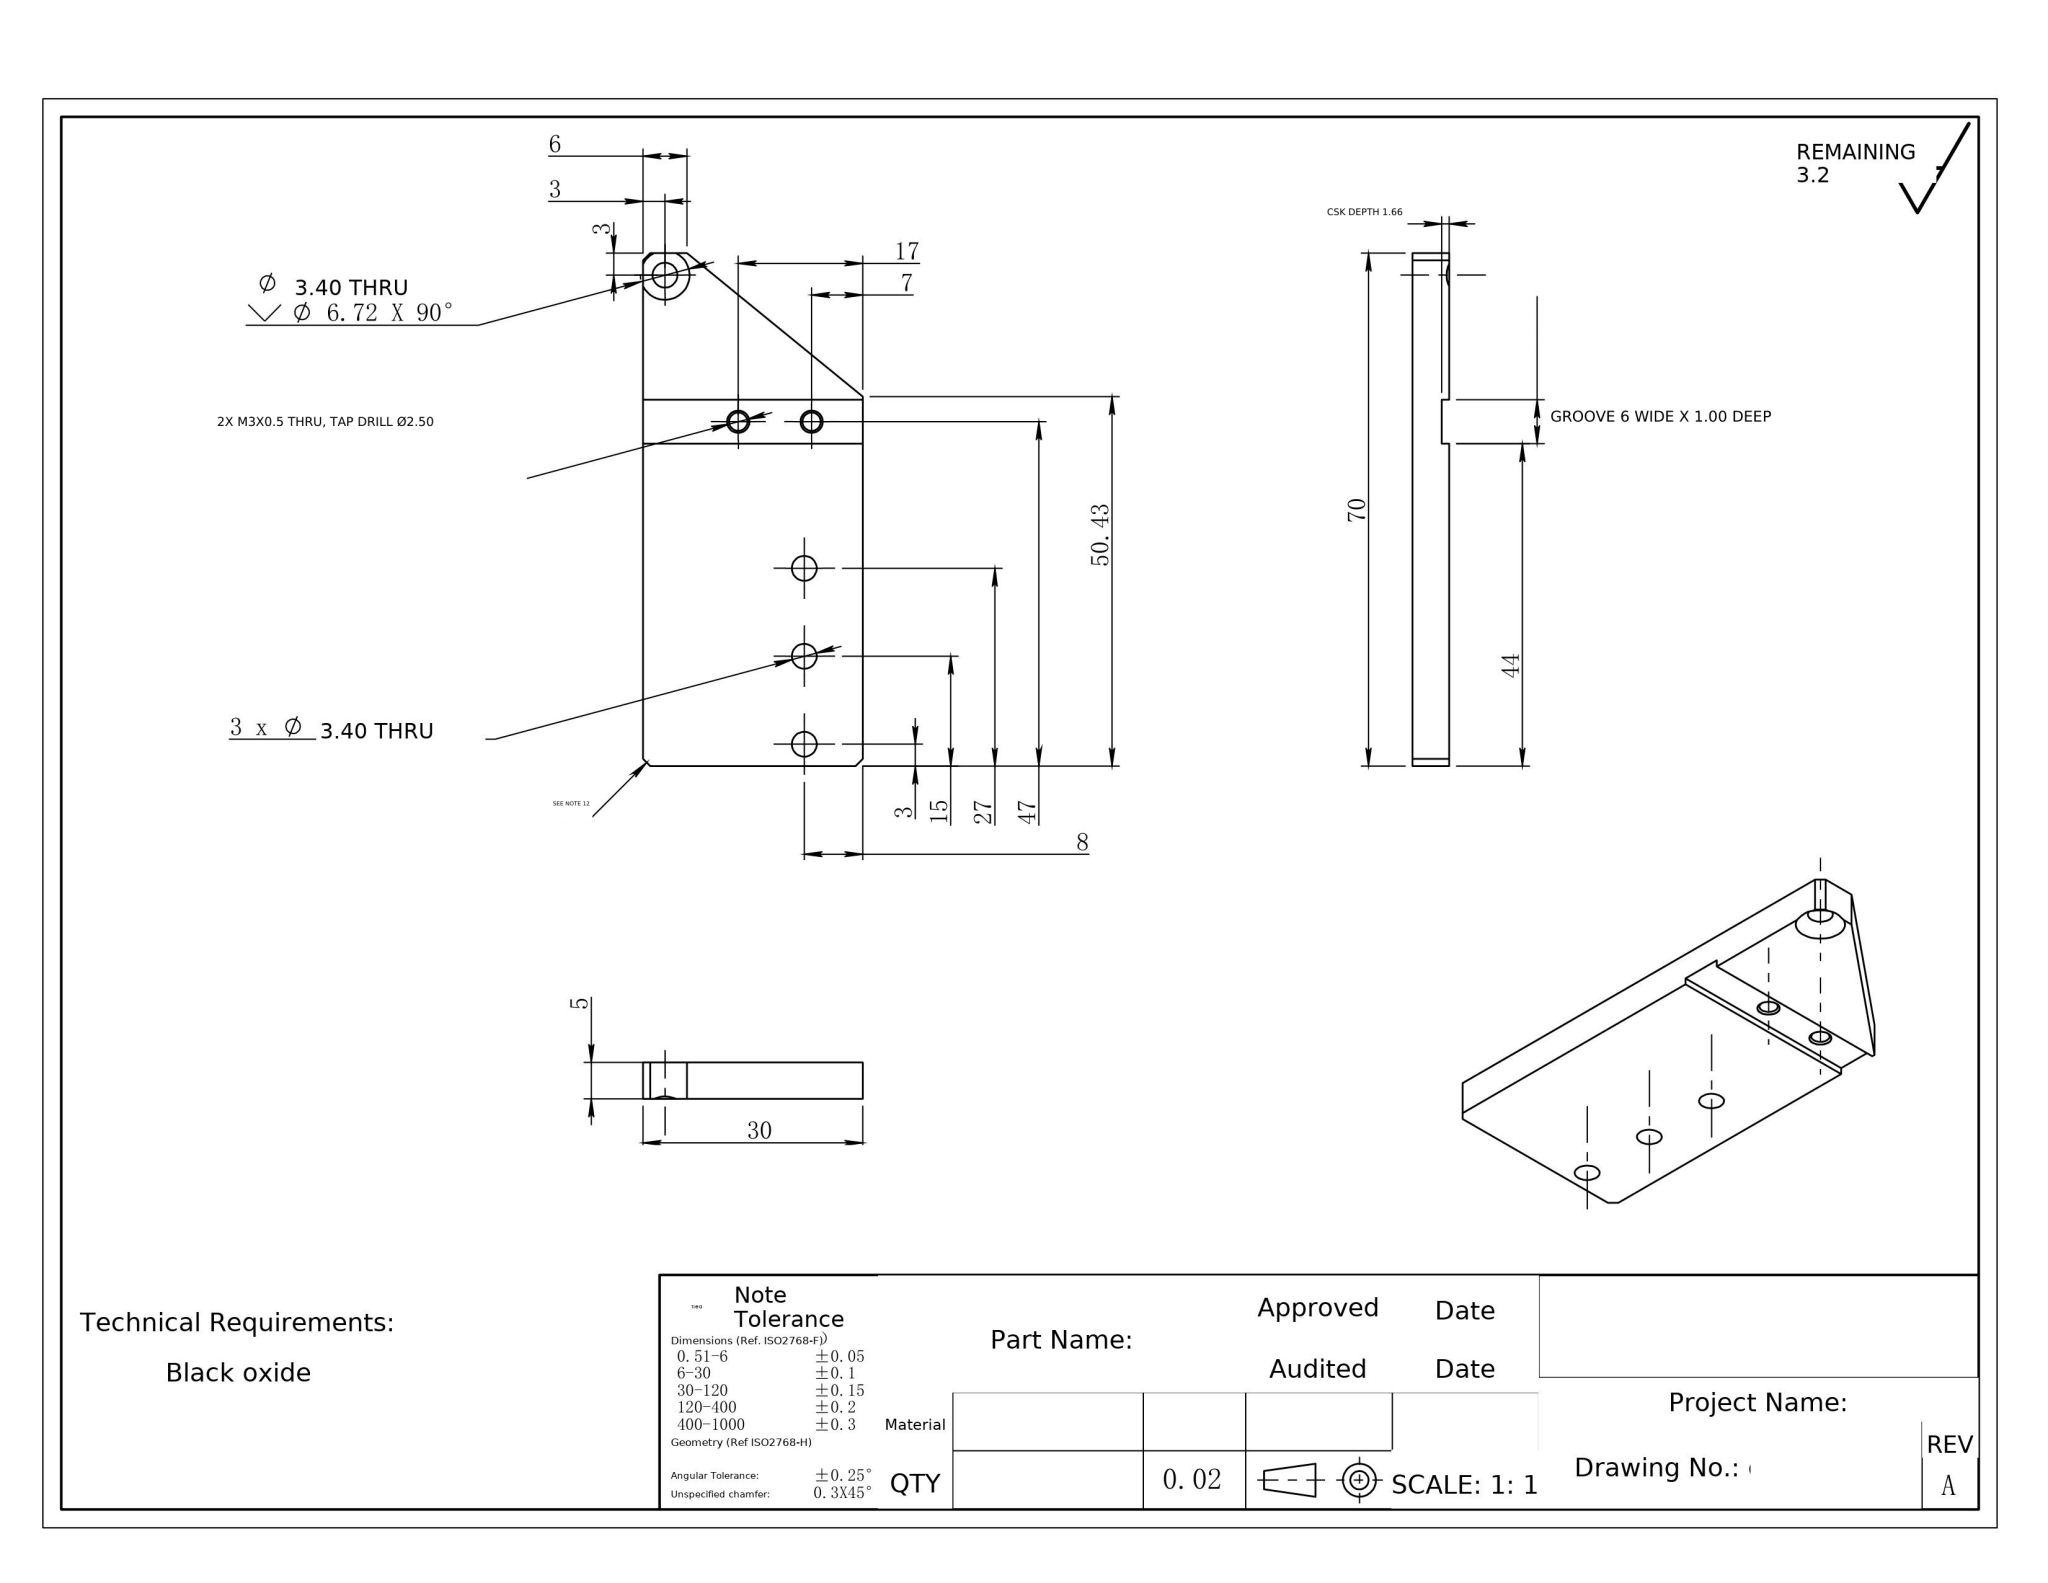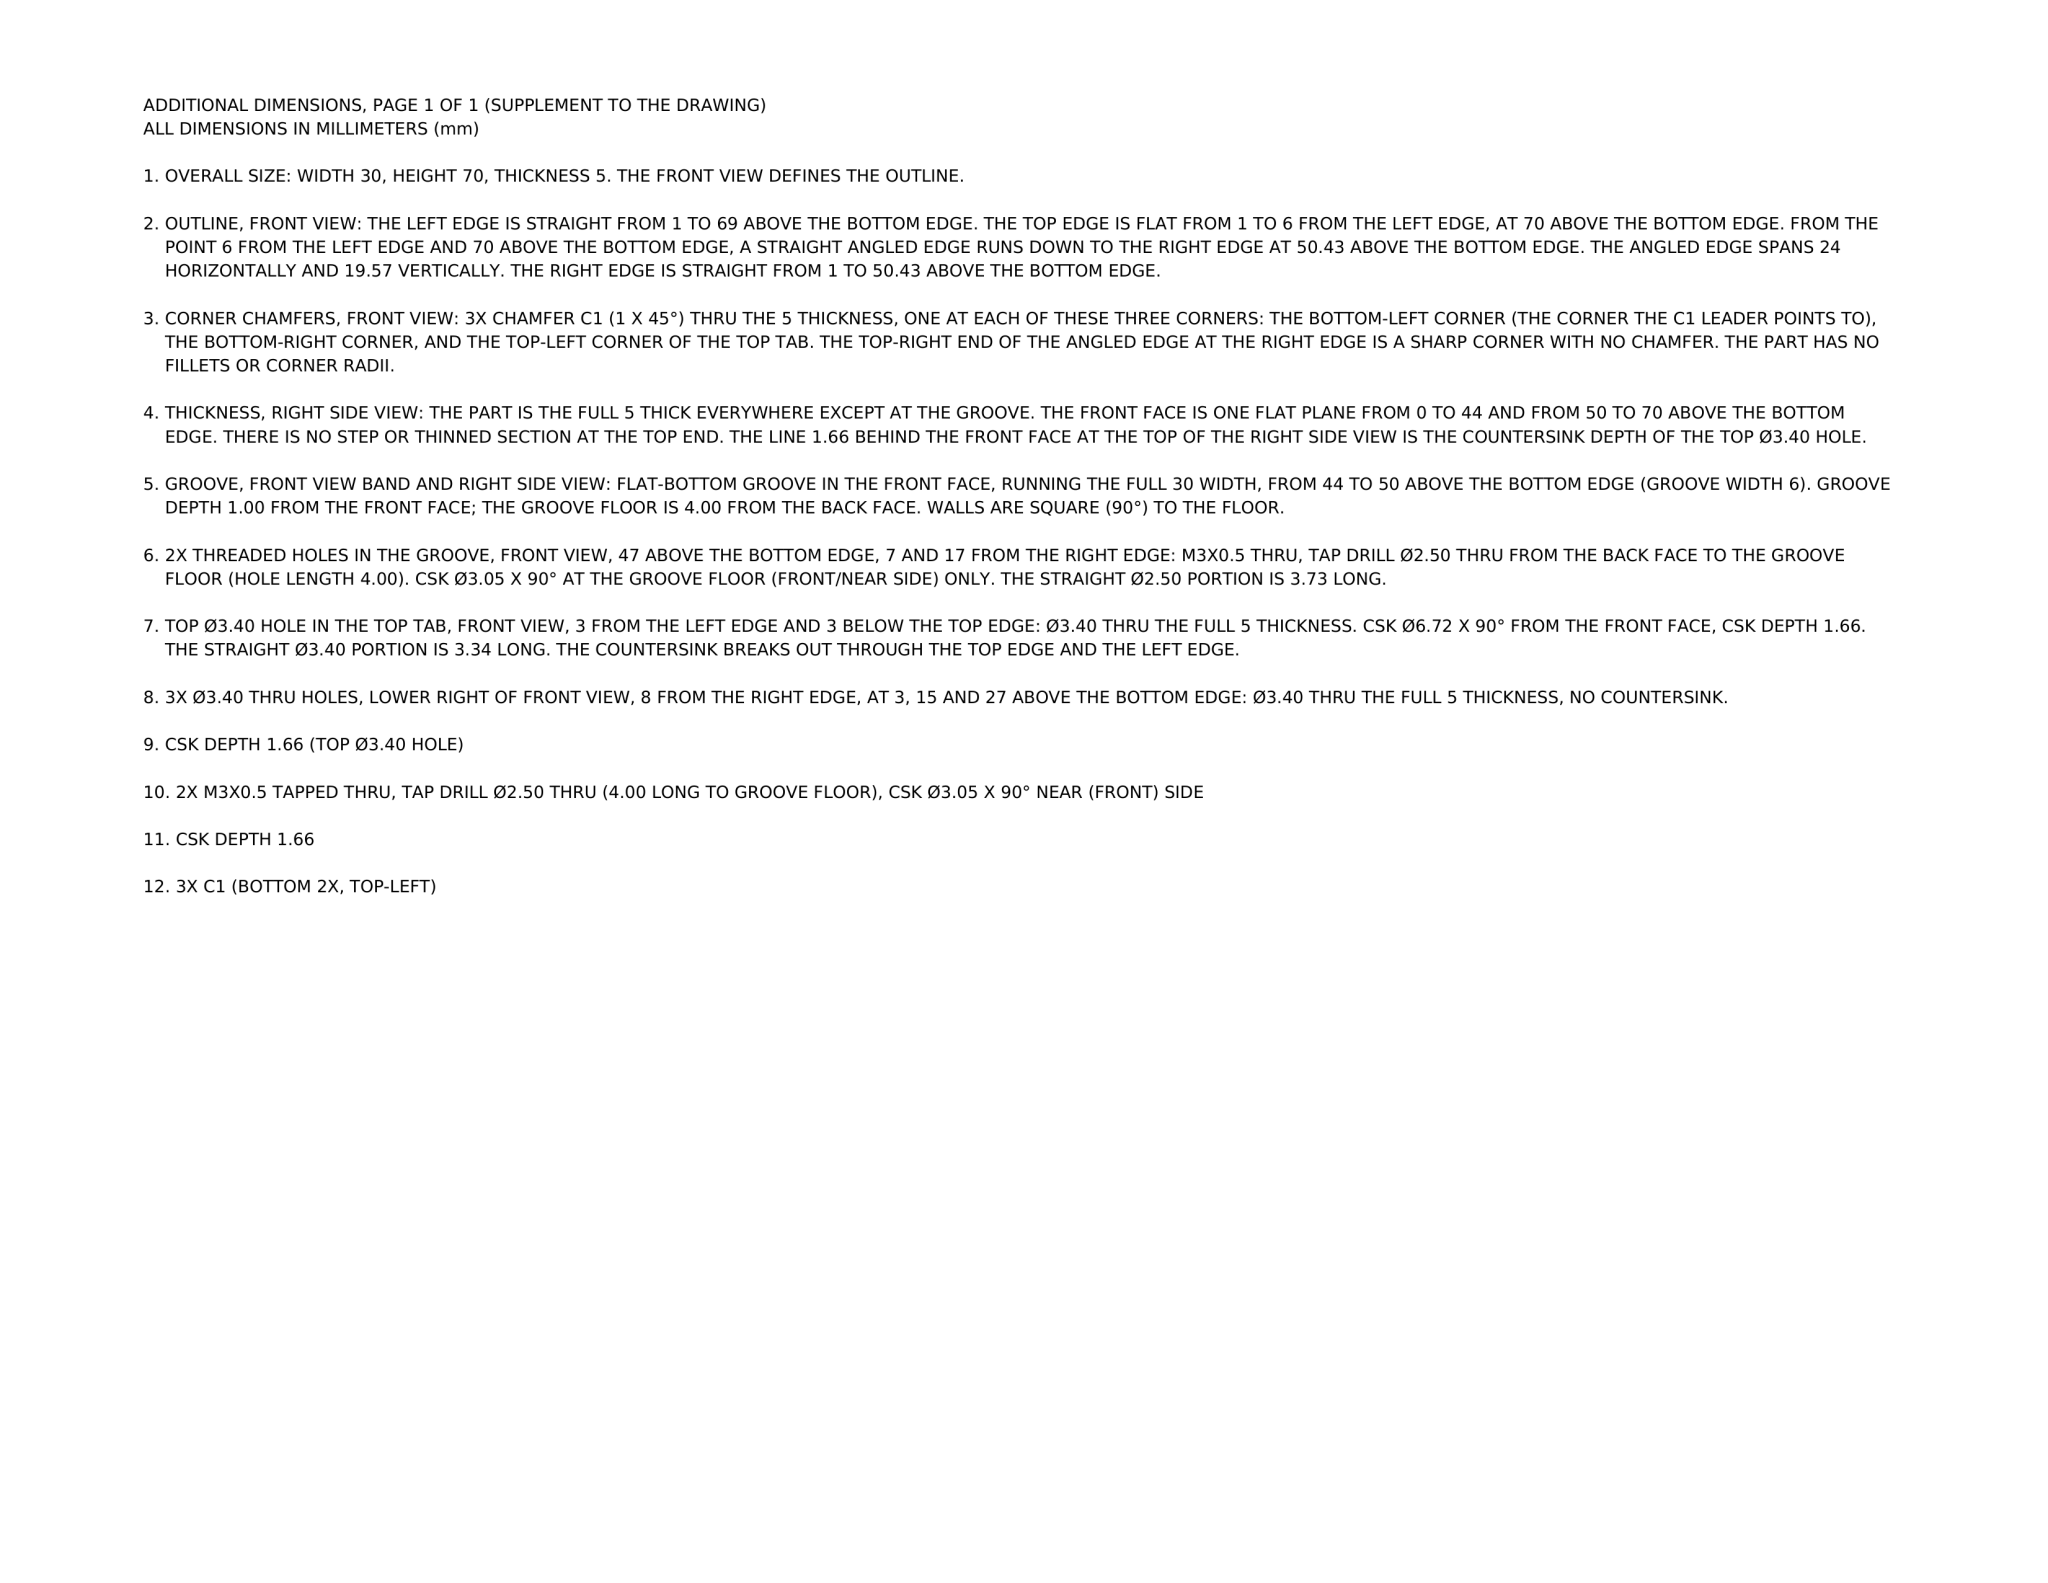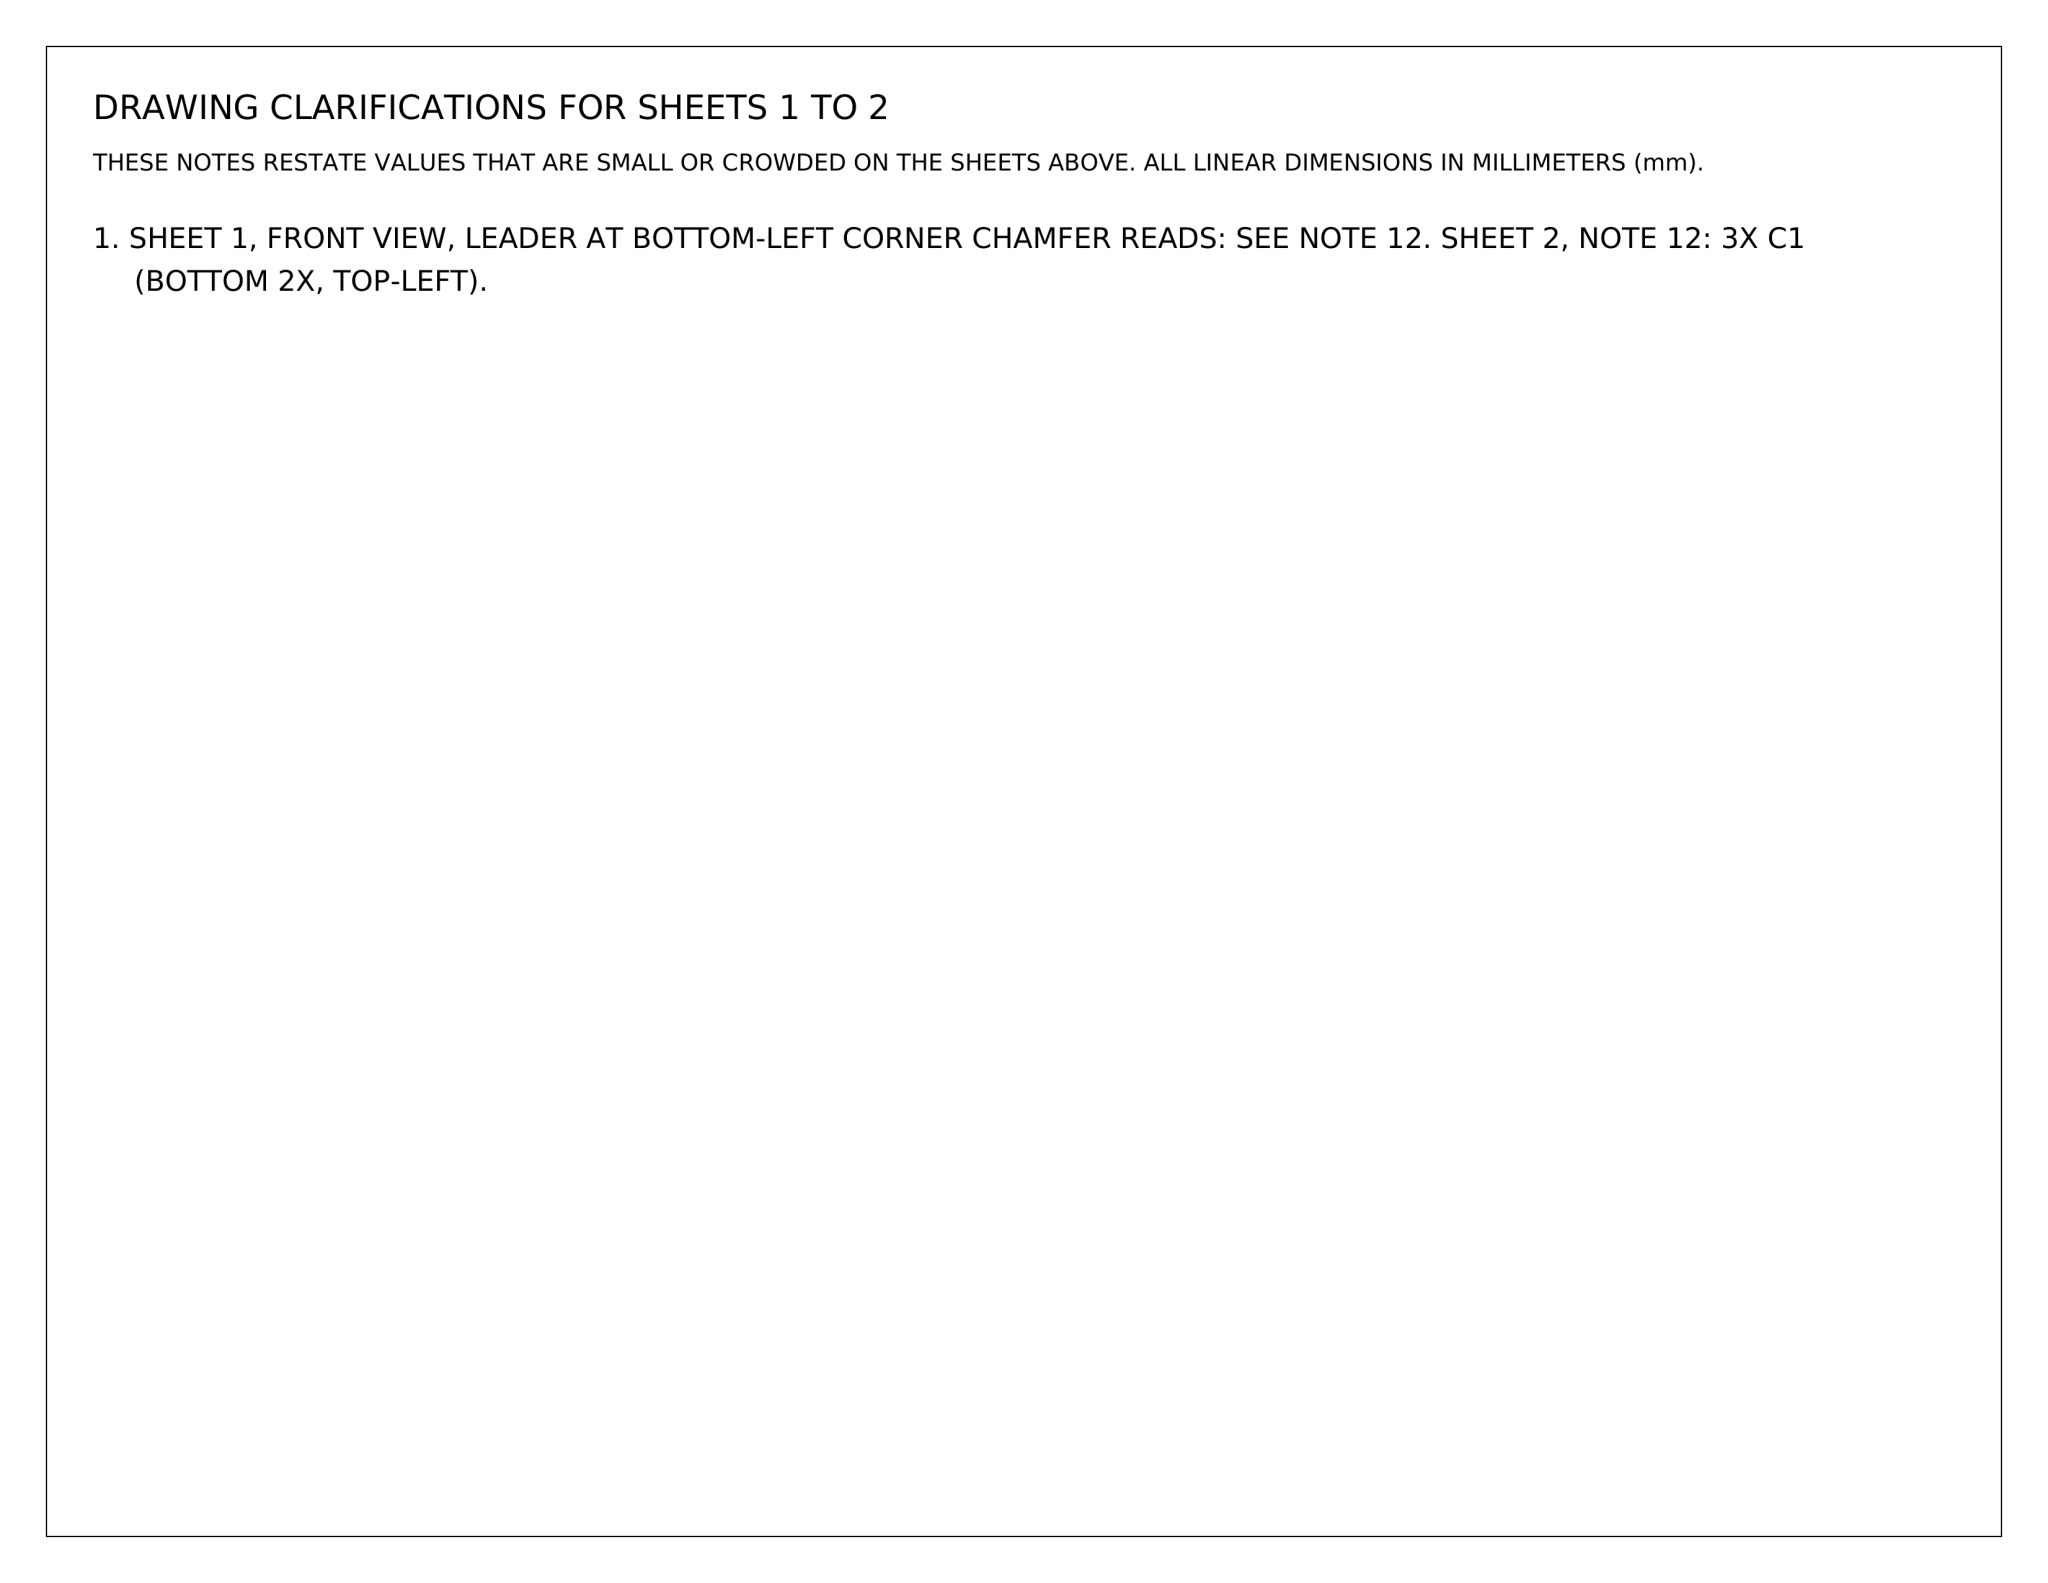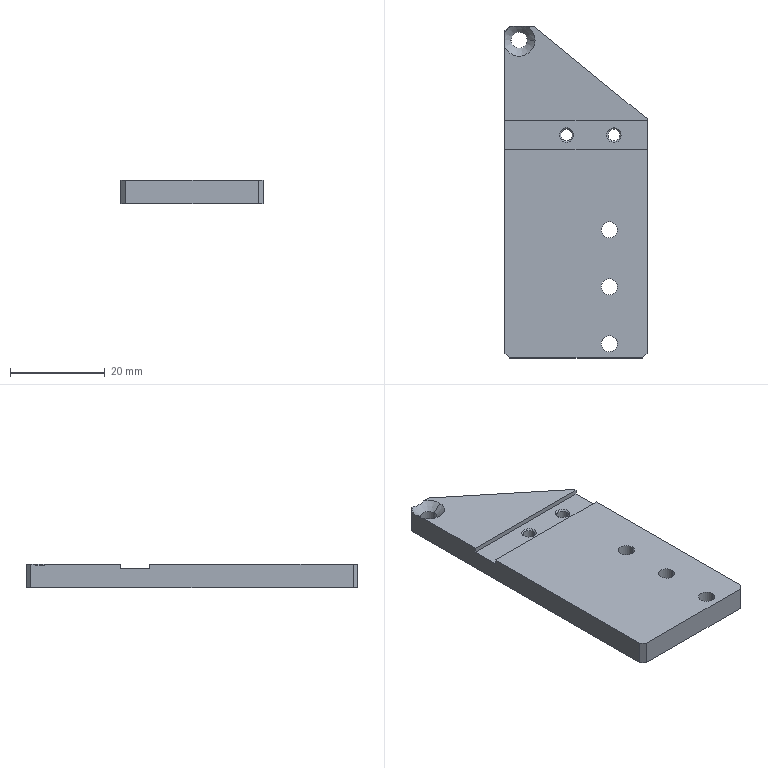Part | NX | mm | 1 solid | 33 faces | box 30 x 70 x 5 mm | volume 8898 mm3 | plane 15 | cylinder 12 | cone 6 | commonest cylinder face diameters 3.4 x8 2.5 x4